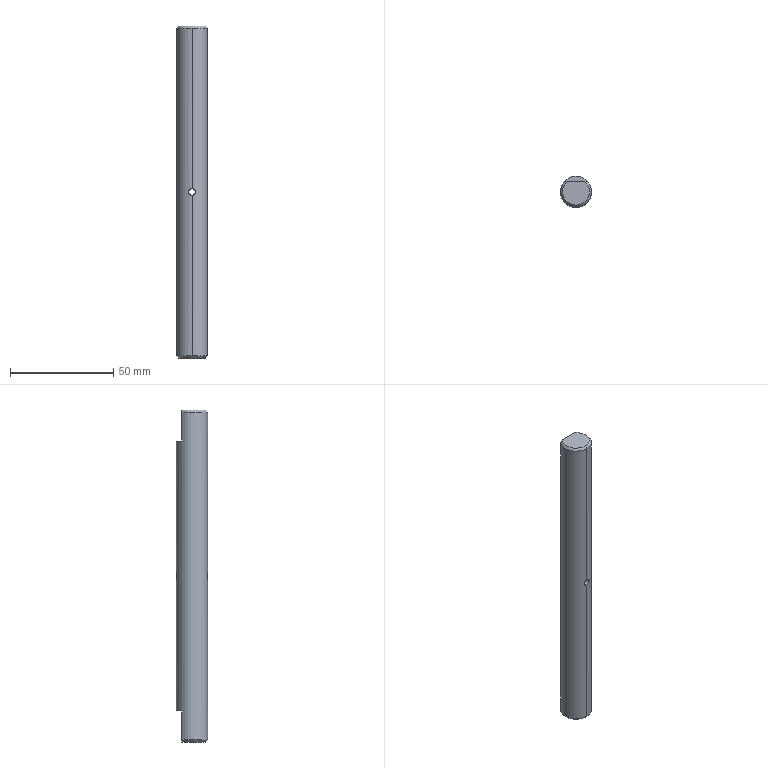Component | SolidWorks | Roller-2-1_XT-1-07-2-1 | 1 solid | 13 faces | box 15 x 15 x 160.5 mm | volume 27621 mm3 | plane 6 | cylinder 4 | cone 3 | commonest cylinder face diameters 3.3 x2 15 x2
STEP:
#1=COLOUR_RGB('',0.7922,0.8196,0.9333);
#2=FILL_AREA_STYLE_COLOUR('',#1);
#3=FILL_AREA_STYLE('',(#2));
#4=SURFACE_STYLE_FILL_AREA(#3);
#5=SURFACE_SIDE_STYLE('',(#4));
#6=SURFACE_STYLE_USAGE(.BOTH.,#5);
#7=PRESENTATION_STYLE_ASSIGNMENT((#6));
#8=CARTESIAN_POINT('',(9.421,3.972,-2.799));
#9=VERTEX_POINT('',#8);
#10=CARTESIAN_POINT('',(9.421,3.972,-2.929));
#11=VERTEX_POINT('',#10);
#12=CARTESIAN_POINT('',(9.421,3.972,-2.799));
#13=CARTESIAN_POINT('',(9.429,3.972,-2.799));
#14=CARTESIAN_POINT('',(9.438,3.972,-2.801));
#15=CARTESIAN_POINT('',(9.449,3.973,-2.806));
#16=CARTESIAN_POINT('',(9.453,3.974,-2.808));
#17=CARTESIAN_POINT('',(9.46,3.974,-2.813));
#18=CARTESIAN_POINT('',(9.464,3.975,-2.815));
#19=CARTESIAN_POINT('',(9.47,3.976,-2.821));
#20=CARTESIAN_POINT('',(9.472,3.976,-2.825));
#21=CARTESIAN_POINT('',(9.477,3.977,-2.832));
#22=CARTESIAN_POINT('',(9.479,3.978,-2.835));
#23=CARTESIAN_POINT('',(9.484,3.979,-2.847));
#24=CARTESIAN_POINT('',(9.486,3.979,-2.856));
#25=CARTESIAN_POINT('',(9.486,3.979,-2.868));
#26=CARTESIAN_POINT('',(9.485,3.979,-2.873));
#27=CARTESIAN_POINT('',(9.483,3.979,-2.881));
#28=CARTESIAN_POINT('',(9.482,3.978,-2.885));
#29=CARTESIAN_POINT('',(9.477,3.977,-2.897));
#30=CARTESIAN_POINT('',(9.473,3.976,-2.904));
#31=CARTESIAN_POINT('',(9.461,3.975,-2.916));
#32=CARTESIAN_POINT('',(9.453,3.974,-2.921));
#33=CARTESIAN_POINT('',(9.442,3.973,-2.926));
#34=CARTESIAN_POINT('',(9.438,3.972,-2.927));
#35=CARTESIAN_POINT('',(9.429,3.972,-2.929));
#36=CARTESIAN_POINT('',(9.425,3.972,-2.929));
#37=CARTESIAN_POINT('',(9.421,3.972,-2.929));
#38=B_SPLINE_CURVE_WITH_KNOTS('',3,(#12,#13,#14,#15,#16,#17,#18,#19,#20,#21,#22,#23,#24,#25,#26,#27,#28,#29,#30,#31,#32,#33,#34,#35,#36,#37),.UNSPECIFIED.,.F.,.F.,(4,2,2,2,2,2,2,2,2,2,2,2,4),(0.005175,0.005821,0.006144,0.006468,0.006791,0.007114,0.007761,0.008084,0.008408,0.009054,0.009701,0.01002,0.01035),.UNSPECIFIED.);
#39=EDGE_CURVE('',#9,#11,#38,.T.);
#40=ORIENTED_EDGE('',*,*,#39,.F.);
#41=CARTESIAN_POINT('',(9.421,4.562,-2.799));
#42=VERTEX_POINT('',#41);
#43=CARTESIAN_POINT('',(9.421,4.602,-2.799));
#44=DIRECTION('',(-0.,1.,0.));
#45=VECTOR('',#44,39.37);
#46=LINE('',#43,#45);
#47=EDGE_CURVE('',#9,#42,#46,.T.);
#48=ORIENTED_EDGE('',*,*,#47,.T.);
#49=CARTESIAN_POINT('',(9.421,4.562,-2.929));
#50=VERTEX_POINT('',#49);
#51=CARTESIAN_POINT('',(9.421,4.562,-2.929));
#52=CARTESIAN_POINT('',(9.425,4.562,-2.929));
#53=CARTESIAN_POINT('',(9.429,4.562,-2.929));
#54=CARTESIAN_POINT('',(9.437,4.562,-2.927));
#55=CARTESIAN_POINT('',(9.442,4.562,-2.926));
#56=CARTESIAN_POINT('',(9.449,4.561,-2.923));
#57=CARTESIAN_POINT('',(9.453,4.561,-2.921));
#58=CARTESIAN_POINT('',(9.46,4.56,-2.916));
#59=CARTESIAN_POINT('',(9.464,4.559,-2.913));
#60=CARTESIAN_POINT('',(9.473,4.558,-2.904));
#61=CARTESIAN_POINT('',(9.477,4.557,-2.897));
#62=CARTESIAN_POINT('',(9.484,4.556,-2.881));
#63=CARTESIAN_POINT('',(9.486,4.555,-2.873));
#64=CARTESIAN_POINT('',(9.486,4.555,-2.86));
#65=CARTESIAN_POINT('',(9.485,4.555,-2.856));
#66=CARTESIAN_POINT('',(9.483,4.556,-2.847));
#67=CARTESIAN_POINT('',(9.482,4.556,-2.843));
#68=CARTESIAN_POINT('',(9.477,4.557,-2.831));
#69=CARTESIAN_POINT('',(9.473,4.558,-2.824));
#70=CARTESIAN_POINT('',(9.464,4.559,-2.815));
#71=CARTESIAN_POINT('',(9.46,4.56,-2.813));
#72=CARTESIAN_POINT('',(9.453,4.561,-2.808));
#73=CARTESIAN_POINT('',(9.449,4.561,-2.806));
#74=CARTESIAN_POINT('',(9.442,4.562,-2.803));
#75=CARTESIAN_POINT('',(9.438,4.562,-2.801));
#76=CARTESIAN_POINT('',(9.429,4.562,-2.8));
#77=CARTESIAN_POINT('',(9.425,4.562,-2.799));
#78=CARTESIAN_POINT('',(9.421,4.562,-2.799));
#79=B_SPLINE_CURVE_WITH_KNOTS('',3,(#51,#52,#53,#54,#55,#56,#57,#58,#59,#60,#61,#62,#63,#64,#65,#66,#67,#68,#69,#70,#71,#72,#73,#74,#75,#76,#77,#78),.UNSPECIFIED.,.F.,.F.,(4,2,2,2,2,2,2,2,2,2,2,2,2,4),(0.,0.0003234,0.0006468,0.0009702,0.001294,0.00194,0.002587,0.002911,0.003234,0.003881,0.004204,0.004528,0.004851,0.005175),.UNSPECIFIED.);
#80=EDGE_CURVE('',#50,#42,#79,.T.);
#81=ORIENTED_EDGE('',*,*,#80,.F.);
#82=CARTESIAN_POINT('',(9.421,4.602,-2.929));
#83=DIRECTION('',(-0.,1.,0.));
#84=VECTOR('',#83,39.37);
#85=LINE('',#82,#84);
#86=EDGE_CURVE('',#11,#50,#85,.T.);
#87=ORIENTED_EDGE('',*,*,#86,.F.);
#88=EDGE_LOOP('',(#40,#48,#81,#87));
#89=FACE_OUTER_BOUND('',#88,.T.);
#90=CARTESIAN_POINT('',(9.421,4.602,-2.864));
#91=DIRECTION('',(-0.,1.,0.));
#92=DIRECTION('',(0.,0.,-1.));
#93=AXIS2_PLACEMENT_3D('',#90,#91,#92);
#94=CYLINDRICAL_SURFACE('',#93,0.06496);
#95=ADVANCED_FACE('',(#89),#94,.F.);
#96=CARTESIAN_POINT('',(9.421,4.011,0.2953));
#97=VERTEX_POINT('',#96);
#98=CARTESIAN_POINT('',(9.584,4.464,0.2953));
#99=VERTEX_POINT('',#98);
#100=CARTESIAN_POINT('',(9.421,4.267,0.2953));
#101=DIRECTION('',(0.,0.,1.));
#102=DIRECTION('',(0.,1.,0.));
#103=AXIS2_PLACEMENT_3D('',#100,#101,#102);
#104=CIRCLE('',#103,0.2559);
#105=EDGE_CURVE('',#97,#99,#104,.T.);
#106=ORIENTED_EDGE('',*,*,#105,.F.);
#107=CARTESIAN_POINT('',(9.421,3.972,0.2559));
#108=VERTEX_POINT('',#107);
#109=CARTESIAN_POINT('',(9.421,4.011,0.2953));
#110=DIRECTION('',(0.,-0.7071,-0.7071));
#111=VECTOR('',#110,39.37);
#112=LINE('',#109,#111);
#113=EDGE_CURVE('',#97,#108,#112,.T.);
#114=ORIENTED_EDGE('',*,*,#113,.T.);
#115=CARTESIAN_POINT('',(9.641,4.464,0.2559));
#116=VERTEX_POINT('',#115);
#117=CARTESIAN_POINT('',(9.421,4.267,0.2559));
#118=DIRECTION('',(0.,0.,-1.));
#119=DIRECTION('',(0.,1.,0.));
#120=AXIS2_PLACEMENT_3D('',#117,#118,#119);
#121=CIRCLE('',#120,0.2953);
#122=EDGE_CURVE('',#116,#108,#121,.T.);
#123=ORIENTED_EDGE('',*,*,#122,.F.);
#124=CARTESIAN_POINT('',(9.584,4.464,0.2953));
#125=CARTESIAN_POINT('',(9.603,4.464,0.2829));
#126=CARTESIAN_POINT('',(9.622,4.464,0.2696));
#127=CARTESIAN_POINT('',(9.641,4.464,0.2559));
#128=B_SPLINE_CURVE_WITH_KNOTS('',3,(#124,#125,#126,#127),.UNSPECIFIED.,.F.,.F.,(4,4),(0.,0.001751),.UNSPECIFIED.);
#129=EDGE_CURVE('',#99,#116,#128,.T.);
#130=ORIENTED_EDGE('',*,*,#129,.F.);
#131=EDGE_LOOP('',(#106,#114,#123,#130));
#132=FACE_OUTER_BOUND('',#131,.T.);
#133=CARTESIAN_POINT('',(9.421,4.267,0.2953));
#134=DIRECTION('',(0.,0.,-1.));
#135=DIRECTION('',(0.,-1.,0.));
#136=AXIS2_PLACEMENT_3D('',#133,#134,#135);
#137=CONICAL_SURFACE('',#136,0.2559,0.7854);
#138=ADVANCED_FACE('',(#132),#137,.T.);
#139=CARTESIAN_POINT('',(9.201,4.464,-0.2953));
#140=VERTEX_POINT('',#139);
#141=CARTESIAN_POINT('',(9.421,4.562,-0.2953));
#142=VERTEX_POINT('',#141);
#143=CARTESIAN_POINT('',(9.421,4.267,-0.2953));
#144=DIRECTION('',(0.,0.,-1.));
#145=DIRECTION('',(0.,-1.,0.));
#146=AXIS2_PLACEMENT_3D('',#143,#144,#145);
#147=CIRCLE('',#146,0.2953);
#148=EDGE_CURVE('',#140,#142,#147,.T.);
#149=ORIENTED_EDGE('',*,*,#148,.T.);
#150=CARTESIAN_POINT('',(9.421,4.562,0.2953));
#151=DIRECTION('',(0.,0.,-1.));
#152=VECTOR('',#151,39.37);
#153=LINE('',#150,#152);
#154=EDGE_CURVE('',#142,#42,#153,.T.);
#155=ORIENTED_EDGE('',*,*,#154,.T.);
#156=CARTESIAN_POINT('',(9.421,4.562,-2.799));
#157=CARTESIAN_POINT('',(9.412,4.562,-2.799));
#158=CARTESIAN_POINT('',(9.404,4.562,-2.801));
#159=CARTESIAN_POINT('',(9.392,4.561,-2.806));
#160=CARTESIAN_POINT('',(9.388,4.561,-2.808));
#161=CARTESIAN_POINT('',(9.381,4.56,-2.813));
#162=CARTESIAN_POINT('',(9.378,4.559,-2.815));
#163=CARTESIAN_POINT('',(9.372,4.558,-2.821));
#164=CARTESIAN_POINT('',(9.369,4.558,-2.825));
#165=CARTESIAN_POINT('',(9.364,4.557,-2.832));
#166=CARTESIAN_POINT('',(9.362,4.557,-2.835));
#167=CARTESIAN_POINT('',(9.357,4.556,-2.847));
#168=CARTESIAN_POINT('',(9.356,4.555,-2.856));
#169=CARTESIAN_POINT('',(9.356,4.555,-2.868));
#170=CARTESIAN_POINT('',(9.356,4.555,-2.873));
#171=CARTESIAN_POINT('',(9.358,4.556,-2.881));
#172=CARTESIAN_POINT('',(9.359,4.556,-2.885));
#173=CARTESIAN_POINT('',(9.364,4.557,-2.897));
#174=CARTESIAN_POINT('',(9.369,4.558,-2.904));
#175=CARTESIAN_POINT('',(9.381,4.56,-2.916));
#176=CARTESIAN_POINT('',(9.388,4.561,-2.921));
#177=CARTESIAN_POINT('',(9.4,4.562,-2.926));
#178=CARTESIAN_POINT('',(9.404,4.562,-2.927));
#179=CARTESIAN_POINT('',(9.412,4.562,-2.929));
#180=CARTESIAN_POINT('',(9.416,4.562,-2.929));
#181=CARTESIAN_POINT('',(9.421,4.562,-2.929));
#182=B_SPLINE_CURVE_WITH_KNOTS('',3,(#156,#157,#158,#159,#160,#161,#162,#163,#164,#165,#166,#167,#168,#169,#170,#171,#172,#173,#174,#175,#176,#177,#178,#179,#180,#181),.UNSPECIFIED.,.F.,.F.,(4,2,2,2,2,2,2,2,2,2,2,2,4),(0.005175,0.005821,0.006144,0.006468,0.006791,0.007114,0.007761,0.008084,0.008408,0.009054,0.009701,0.01002,0.01035),.UNSPECIFIED.);
#183=EDGE_CURVE('',#42,#50,#182,.T.);
#184=ORIENTED_EDGE('',*,*,#183,.T.);
#185=CARTESIAN_POINT('',(9.421,4.562,-5.433));
#186=VERTEX_POINT('',#185);
#187=CARTESIAN_POINT('',(9.421,4.562,0.2953));
#188=DIRECTION('',(0.,0.,-1.));
#189=VECTOR('',#188,39.37);
#190=LINE('',#187,#189);
#191=EDGE_CURVE('',#50,#186,#190,.T.);
#192=ORIENTED_EDGE('',*,*,#191,.T.);
#193=CARTESIAN_POINT('',(9.201,4.464,-5.433));
#194=VERTEX_POINT('',#193);
#195=CARTESIAN_POINT('',(9.421,4.267,-5.433));
#196=DIRECTION('',(0.,0.,1.));
#197=DIRECTION('',(0.,1.,0.));
#198=AXIS2_PLACEMENT_3D('',#195,#196,#197);
#199=CIRCLE('',#198,0.2953);
#200=EDGE_CURVE('',#186,#194,#199,.T.);
#201=ORIENTED_EDGE('',*,*,#200,.T.);
#202=CARTESIAN_POINT('',(9.201,4.464,-5.984));
#203=VERTEX_POINT('',#202);
#204=CARTESIAN_POINT('',(9.201,4.464,-5.433));
#205=DIRECTION('',(0.,0.,-1.));
#206=VECTOR('',#205,39.37);
#207=LINE('',#204,#206);
#208=EDGE_CURVE('',#194,#203,#207,.T.);
#209=ORIENTED_EDGE('',*,*,#208,.T.);
#210=CARTESIAN_POINT('',(9.421,3.972,-5.984));
#211=VERTEX_POINT('',#210);
#212=CARTESIAN_POINT('',(9.421,4.267,-5.984));
#213=DIRECTION('',(0.,0.,1.));
#214=DIRECTION('',(0.,1.,0.));
#215=AXIS2_PLACEMENT_3D('',#212,#213,#214);
#216=CIRCLE('',#215,0.2953);
#217=EDGE_CURVE('',#203,#211,#216,.T.);
#218=ORIENTED_EDGE('',*,*,#217,.T.);
#219=CARTESIAN_POINT('',(9.421,3.972,0.2953));
#220=DIRECTION('',(0.,0.,-1.));
#221=VECTOR('',#220,39.37);
#222=LINE('',#219,#221);
#223=EDGE_CURVE('',#11,#211,#222,.T.);
#224=ORIENTED_EDGE('',*,*,#223,.F.);
#225=CARTESIAN_POINT('',(9.421,3.972,-2.929));
#226=CARTESIAN_POINT('',(9.416,3.972,-2.929));
#227=CARTESIAN_POINT('',(9.412,3.972,-2.929));
#228=CARTESIAN_POINT('',(9.404,3.972,-2.927));
#229=CARTESIAN_POINT('',(9.4,3.973,-2.926));
#230=CARTESIAN_POINT('',(9.392,3.973,-2.923));
#231=CARTESIAN_POINT('',(9.388,3.974,-2.921));
#232=CARTESIAN_POINT('',(9.381,3.974,-2.916));
#233=CARTESIAN_POINT('',(9.378,3.975,-2.913));
#234=CARTESIAN_POINT('',(9.369,3.976,-2.904));
#235=CARTESIAN_POINT('',(9.364,3.977,-2.897));
#236=CARTESIAN_POINT('',(9.357,3.979,-2.881));
#237=CARTESIAN_POINT('',(9.356,3.979,-2.873));
#238=CARTESIAN_POINT('',(9.356,3.979,-2.86));
#239=CARTESIAN_POINT('',(9.356,3.979,-2.856));
#240=CARTESIAN_POINT('',(9.358,3.979,-2.847));
#241=CARTESIAN_POINT('',(9.359,3.978,-2.843));
#242=CARTESIAN_POINT('',(9.364,3.977,-2.831));
#243=CARTESIAN_POINT('',(9.369,3.976,-2.824));
#244=CARTESIAN_POINT('',(9.378,3.975,-2.815));
#245=CARTESIAN_POINT('',(9.381,3.974,-2.813));
#246=CARTESIAN_POINT('',(9.388,3.974,-2.808));
#247=CARTESIAN_POINT('',(9.392,3.973,-2.806));
#248=CARTESIAN_POINT('',(9.4,3.973,-2.803));
#249=CARTESIAN_POINT('',(9.404,3.972,-2.801));
#250=CARTESIAN_POINT('',(9.412,3.972,-2.8));
#251=CARTESIAN_POINT('',(9.416,3.972,-2.799));
#252=CARTESIAN_POINT('',(9.421,3.972,-2.799));
#253=B_SPLINE_CURVE_WITH_KNOTS('',3,(#225,#226,#227,#228,#229,#230,#231,#232,#233,#234,#235,#236,#237,#238,#239,#240,#241,#242,#243,#244,#245,#246,#247,#248,#249,#250,#251,#252),.UNSPECIFIED.,.F.,.F.,(4,2,2,2,2,2,2,2,2,2,2,2,2,4),(0.,0.0003234,0.0006468,0.0009702,0.001294,0.00194,0.002587,0.002911,0.003234,0.003881,0.004204,0.004528,0.004851,0.005175),.UNSPECIFIED.);
#254=EDGE_CURVE('',#11,#9,#253,.T.);
#255=ORIENTED_EDGE('',*,*,#254,.T.);
#256=CARTESIAN_POINT('',(9.421,3.972,0.2953));
#257=DIRECTION('',(0.,0.,-1.));
#258=VECTOR('',#257,39.37);
#259=LINE('',#256,#258);
#260=EDGE_CURVE('',#108,#9,#259,.T.);
#261=ORIENTED_EDGE('',*,*,#260,.F.);
#262=CARTESIAN_POINT('',(9.201,4.464,0.2559));
#263=VERTEX_POINT('',#262);
#264=CARTESIAN_POINT('',(9.421,4.267,0.2559));
#265=DIRECTION('',(0.,0.,-1.));
#266=DIRECTION('',(0.,1.,0.));
#267=AXIS2_PLACEMENT_3D('',#264,#265,#266);
#268=CIRCLE('',#267,0.2953);
#269=EDGE_CURVE('',#108,#263,#268,.T.);
#270=ORIENTED_EDGE('',*,*,#269,.T.);
#271=CARTESIAN_POINT('',(9.201,4.464,-0.2953));
#272=DIRECTION('',(0.,0.,1.));
#273=VECTOR('',#272,39.37);
#274=LINE('',#271,#273);
#275=EDGE_CURVE('',#140,#263,#274,.T.);
#276=ORIENTED_EDGE('',*,*,#275,.F.);
#277=EDGE_LOOP('',(#149,#155,#184,#192,#201,#209,#218,#224,#255,#261,#270,#276));
#278=FACE_OUTER_BOUND('',#277,.T.);
#279=CARTESIAN_POINT('',(9.421,4.267,0.2953));
#280=DIRECTION('',(0.,0.,-1.));
#281=DIRECTION('',(0.,-1.,0.));
#282=AXIS2_PLACEMENT_3D('',#279,#280,#281);
#283=CYLINDRICAL_SURFACE('',#282,0.2953);
#284=ADVANCED_FACE('',(#278),#283,.T.);
#285=ORIENTED_EDGE('',*,*,#154,.F.);
#286=CARTESIAN_POINT('',(9.641,4.464,-0.2953));
#287=VERTEX_POINT('',#286);
#288=CARTESIAN_POINT('',(9.421,4.267,-0.2953));
#289=DIRECTION('',(0.,0.,-1.));
#290=DIRECTION('',(0.,-1.,0.));
#291=AXIS2_PLACEMENT_3D('',#288,#289,#290);
#292=CIRCLE('',#291,0.2953);
#293=EDGE_CURVE('',#142,#287,#292,.T.);
#294=ORIENTED_EDGE('',*,*,#293,.T.);
#295=CARTESIAN_POINT('',(9.641,4.464,-0.2953));
#296=DIRECTION('',(0.,0.,1.));
#297=VECTOR('',#296,39.37);
#298=LINE('',#295,#297);
#299=EDGE_CURVE('',#287,#116,#298,.T.);
#300=ORIENTED_EDGE('',*,*,#299,.T.);
#301=ORIENTED_EDGE('',*,*,#122,.T.);
#302=ORIENTED_EDGE('',*,*,#260,.T.);
#303=ORIENTED_EDGE('',*,*,#39,.T.);
#304=ORIENTED_EDGE('',*,*,#223,.T.);
#305=CARTESIAN_POINT('',(9.641,4.464,-5.984));
#306=VERTEX_POINT('',#305);
#307=CARTESIAN_POINT('',(9.421,4.267,-5.984));
#308=DIRECTION('',(0.,0.,1.));
#309=DIRECTION('',(0.,1.,0.));
#310=AXIS2_PLACEMENT_3D('',#307,#308,#309);
#311=CIRCLE('',#310,0.2953);
#312=EDGE_CURVE('',#211,#306,#311,.T.);
#313=ORIENTED_EDGE('',*,*,#312,.T.);
#314=CARTESIAN_POINT('',(9.641,4.464,-5.433));
#315=VERTEX_POINT('',#314);
#316=CARTESIAN_POINT('',(9.641,4.464,-5.433));
#317=DIRECTION('',(0.,0.,-1.));
#318=VECTOR('',#317,39.37);
#319=LINE('',#316,#318);
#320=EDGE_CURVE('',#315,#306,#319,.T.);
#321=ORIENTED_EDGE('',*,*,#320,.F.);
#322=CARTESIAN_POINT('',(9.421,4.267,-5.433));
#323=DIRECTION('',(0.,0.,1.));
#324=DIRECTION('',(0.,1.,0.));
#325=AXIS2_PLACEMENT_3D('',#322,#323,#324);
#326=CIRCLE('',#325,0.2953);
#327=EDGE_CURVE('',#315,#186,#326,.T.);
#328=ORIENTED_EDGE('',*,*,#327,.T.);
#329=ORIENTED_EDGE('',*,*,#191,.F.);
#330=ORIENTED_EDGE('',*,*,#80,.T.);
#331=EDGE_LOOP('',(#285,#294,#300,#301,#302,#303,#304,#313,#321,#328,#329,#330));
#332=FACE_OUTER_BOUND('',#331,.T.);
#333=CARTESIAN_POINT('',(9.421,4.267,0.2953));
#334=DIRECTION('',(0.,0.,-1.));
#335=DIRECTION('',(0.,-1.,0.));
#336=AXIS2_PLACEMENT_3D('',#333,#334,#335);
#337=CYLINDRICAL_SURFACE('',#336,0.2953);
#338=ADVANCED_FACE('',(#332),#337,.T.);
#339=CARTESIAN_POINT('',(9.257,4.464,0.2953));
#340=VERTEX_POINT('',#339);
#341=CARTESIAN_POINT('',(9.201,4.464,0.2953));
#342=DIRECTION('',(1.,0.,0.));
#343=VECTOR('',#342,39.37);
#344=LINE('',#341,#343);
#345=EDGE_CURVE('',#340,#99,#344,.T.);
#346=ORIENTED_EDGE('',*,*,#345,.F.);
#347=CARTESIAN_POINT('',(9.421,4.267,0.2953));
#348=DIRECTION('',(0.,0.,1.));
#349=DIRECTION('',(0.,1.,0.));
#350=AXIS2_PLACEMENT_3D('',#347,#348,#349);
#351=CIRCLE('',#350,0.2559);
#352=EDGE_CURVE('',#340,#97,#351,.T.);
#353=ORIENTED_EDGE('',*,*,#352,.T.);
#354=ORIENTED_EDGE('',*,*,#105,.T.);
#355=EDGE_LOOP('',(#346,#353,#354));
#356=FACE_OUTER_BOUND('',#355,.T.);
#357=CARTESIAN_POINT('',(9.421,4.267,0.2953));
#358=DIRECTION('',(0.,0.,1.));
#359=DIRECTION('',(-0.,1.,0.));
#360=AXIS2_PLACEMENT_3D('',#357,#358,#359);
#361=PLANE('',#360);
#362=ADVANCED_FACE('',(#356),#361,.T.);
#363=CARTESIAN_POINT('',(9.584,4.464,-6.024));
#364=VERTEX_POINT('',#363);
#365=CARTESIAN_POINT('',(9.257,4.464,-6.024));
#366=VERTEX_POINT('',#365);
#367=CARTESIAN_POINT('',(9.201,4.464,-6.024));
#368=DIRECTION('',(-1.,-0.,0.));
#369=VECTOR('',#368,39.37);
#370=LINE('',#367,#369);
#371=EDGE_CURVE('',#364,#366,#370,.T.);
#372=ORIENTED_EDGE('',*,*,#371,.F.);
#373=CARTESIAN_POINT('',(9.421,4.267,-6.024));
#374=DIRECTION('',(0.,0.,-1.));
#375=DIRECTION('',(0.,1.,0.));
#376=AXIS2_PLACEMENT_3D('',#373,#374,#375);
#377=CIRCLE('',#376,0.2559);
#378=EDGE_CURVE('',#364,#366,#377,.T.);
#379=ORIENTED_EDGE('',*,*,#378,.T.);
#380=EDGE_LOOP('',(#372,#379));
#381=FACE_OUTER_BOUND('',#380,.T.);
#382=CARTESIAN_POINT('',(9.421,4.267,-6.024));
#383=DIRECTION('',(0.,0.,1.));
#384=DIRECTION('',(-0.,1.,0.));
#385=AXIS2_PLACEMENT_3D('',#382,#383,#384);
#386=PLANE('',#385);
#387=ADVANCED_FACE('',(#381),#386,.F.);
#388=CARTESIAN_POINT('',(9.201,4.464,-0.2953));
#389=DIRECTION('',(1.,0.,0.));
#390=VECTOR('',#389,39.37);
#391=LINE('',#388,#390);
#392=EDGE_CURVE('',#140,#287,#391,.T.);
#393=ORIENTED_EDGE('',*,*,#392,.T.);
#394=ORIENTED_EDGE('',*,*,#293,.F.);
#395=ORIENTED_EDGE('',*,*,#148,.F.);
#396=EDGE_LOOP('',(#393,#394,#395));
#397=FACE_OUTER_BOUND('',#396,.T.);
#398=CARTESIAN_POINT('',(9.201,4.728,-0.2953));
#399=DIRECTION('',(0.,0.,-1.));
#400=DIRECTION('',(0.,-1.,0.));
#401=AXIS2_PLACEMENT_3D('',#398,#399,#400);
#402=PLANE('',#401);
#403=ADVANCED_FACE('',(#397),#402,.F.);
#404=ORIENTED_EDGE('',*,*,#345,.T.);
#405=ORIENTED_EDGE('',*,*,#129,.T.);
#406=ORIENTED_EDGE('',*,*,#299,.F.);
#407=ORIENTED_EDGE('',*,*,#392,.F.);
#408=ORIENTED_EDGE('',*,*,#275,.T.);
#409=CARTESIAN_POINT('',(9.201,4.464,0.2559));
#410=CARTESIAN_POINT('',(9.219,4.464,0.2696));
#411=CARTESIAN_POINT('',(9.238,4.464,0.2829));
#412=CARTESIAN_POINT('',(9.257,4.464,0.2953));
#413=B_SPLINE_CURVE_WITH_KNOTS('',3,(#409,#410,#411,#412),.UNSPECIFIED.,.F.,.F.,(4,4),(0.,0.001751),.UNSPECIFIED.);
#414=EDGE_CURVE('',#263,#340,#413,.T.);
#415=ORIENTED_EDGE('',*,*,#414,.T.);
#416=EDGE_LOOP('',(#404,#405,#406,#407,#408,#415));
#417=FACE_OUTER_BOUND('',#416,.T.);
#418=CARTESIAN_POINT('',(9.201,4.464,-0.2953));
#419=DIRECTION('',(0.,-1.,0.));
#420=DIRECTION('',(0.,0.,1.));
#421=AXIS2_PLACEMENT_3D('',#418,#419,#420);
#422=PLANE('',#421);
#423=ADVANCED_FACE('',(#417),#422,.F.);
#424=CARTESIAN_POINT('',(9.201,4.464,-5.433));
#425=DIRECTION('',(-1.,-0.,0.));
#426=VECTOR('',#425,39.37);
#427=LINE('',#424,#426);
#428=EDGE_CURVE('',#315,#194,#427,.T.);
#429=ORIENTED_EDGE('',*,*,#428,.T.);
#430=ORIENTED_EDGE('',*,*,#200,.F.);
#431=ORIENTED_EDGE('',*,*,#327,.F.);
#432=EDGE_LOOP('',(#429,#430,#431));
#433=FACE_OUTER_BOUND('',#432,.T.);
#434=CARTESIAN_POINT('',(9.201,4.464,-5.433));
#435=DIRECTION('',(0.,0.,1.));
#436=DIRECTION('',(-0.,1.,0.));
#437=AXIS2_PLACEMENT_3D('',#434,#435,#436);
#438=PLANE('',#437);
#439=ADVANCED_FACE('',(#433),#438,.F.);
#440=ORIENTED_EDGE('',*,*,#320,.T.);
#441=CARTESIAN_POINT('',(9.641,4.464,-5.984));
#442=CARTESIAN_POINT('',(9.622,4.464,-5.998));
#443=CARTESIAN_POINT('',(9.603,4.464,-6.011));
#444=CARTESIAN_POINT('',(9.584,4.464,-6.024));
#445=B_SPLINE_CURVE_WITH_KNOTS('',3,(#441,#442,#443,#444),.UNSPECIFIED.,.F.,.F.,(4,4),(0.,0.001751),.UNSPECIFIED.);
#446=EDGE_CURVE('',#306,#364,#445,.T.);
#447=ORIENTED_EDGE('',*,*,#446,.T.);
#448=ORIENTED_EDGE('',*,*,#371,.T.);
#449=CARTESIAN_POINT('',(9.257,4.464,-6.024));
#450=CARTESIAN_POINT('',(9.238,4.464,-6.011));
#451=CARTESIAN_POINT('',(9.219,4.464,-5.998));
#452=CARTESIAN_POINT('',(9.201,4.464,-5.984));
#453=B_SPLINE_CURVE_WITH_KNOTS('',3,(#449,#450,#451,#452),.UNSPECIFIED.,.F.,.F.,(4,4),(0.,0.001751),.UNSPECIFIED.);
#454=EDGE_CURVE('',#366,#203,#453,.T.);
#455=ORIENTED_EDGE('',*,*,#454,.T.);
#456=ORIENTED_EDGE('',*,*,#208,.F.);
#457=ORIENTED_EDGE('',*,*,#428,.F.);
#458=EDGE_LOOP('',(#440,#447,#448,#455,#456,#457));
#459=FACE_OUTER_BOUND('',#458,.T.);
#460=CARTESIAN_POINT('',(9.201,4.464,-5.433));
#461=DIRECTION('',(0.,-1.,0.));
#462=DIRECTION('',(0.,0.,1.));
#463=AXIS2_PLACEMENT_3D('',#460,#461,#462);
#464=PLANE('',#463);
#465=ADVANCED_FACE('',(#459),#464,.F.);
#466=ORIENTED_EDGE('',*,*,#454,.F.);
#467=ORIENTED_EDGE('',*,*,#378,.F.);
#468=ORIENTED_EDGE('',*,*,#446,.F.);
#469=ORIENTED_EDGE('',*,*,#312,.F.);
#470=ORIENTED_EDGE('',*,*,#217,.F.);
#471=EDGE_LOOP('',(#466,#467,#468,#469,#470));
#472=FACE_OUTER_BOUND('',#471,.T.);
#473=CARTESIAN_POINT('',(9.421,4.267,-5.984));
#474=DIRECTION('',(0.,0.,1.));
#475=DIRECTION('',(0.,1.,0.));
#476=AXIS2_PLACEMENT_3D('',#473,#474,#475);
#477=CONICAL_SURFACE('',#476,0.2953,0.7854);
#478=ADVANCED_FACE('',(#472),#477,.T.);
#479=ORIENTED_EDGE('',*,*,#113,.F.);
#480=ORIENTED_EDGE('',*,*,#352,.F.);
#481=ORIENTED_EDGE('',*,*,#414,.F.);
#482=ORIENTED_EDGE('',*,*,#269,.F.);
#483=EDGE_LOOP('',(#479,#480,#481,#482));
#484=FACE_OUTER_BOUND('',#483,.T.);
#485=CARTESIAN_POINT('',(9.421,4.267,0.2953));
#486=DIRECTION('',(0.,0.,-1.));
#487=DIRECTION('',(0.,-1.,0.));
#488=AXIS2_PLACEMENT_3D('',#485,#486,#487);
#489=CONICAL_SURFACE('',#488,0.2559,0.7854);
#490=ADVANCED_FACE('',(#484),#489,.T.);
#491=ORIENTED_EDGE('',*,*,#47,.F.);
#492=ORIENTED_EDGE('',*,*,#254,.F.);
#493=ORIENTED_EDGE('',*,*,#86,.T.);
#494=ORIENTED_EDGE('',*,*,#183,.F.);
#495=EDGE_LOOP('',(#491,#492,#493,#494));
#496=FACE_OUTER_BOUND('',#495,.T.);
#497=CARTESIAN_POINT('',(9.421,4.602,-2.864));
#498=DIRECTION('',(-0.,1.,0.));
#499=DIRECTION('',(0.,0.,-1.));
#500=AXIS2_PLACEMENT_3D('',#497,#498,#499);
#501=CYLINDRICAL_SURFACE('',#500,0.06496);
#502=ADVANCED_FACE('',(#496),#501,.F.);
#503=CLOSED_SHELL('',(#95,#138,#284,#338,#362,#387,#403,#423,#439,#465,#478,#490,#502));
#504=MANIFOLD_SOLID_BREP('',#503);
#505=STYLED_ITEM('',(#7),#504);
#506=(LENGTH_UNIT()NAMED_UNIT(*)SI_UNIT($,.METRE.));
#507=LENGTH_MEASURE_WITH_UNIT(LENGTH_MEASURE(0.0254),#506);
#508=DIMENSIONAL_EXPONENTS(1.,0.,0.,0.,0.,0.,0.);
#509=(CONVERSION_BASED_UNIT('',#507)LENGTH_UNIT()NAMED_UNIT(#508));
#510=UNCERTAINTY_MEASURE_WITH_UNIT(LENGTH_MEASURE(0.00001),#509,'','');
#511=(NAMED_UNIT(*)PLANE_ANGLE_UNIT()SI_UNIT($,.RADIAN.));
#512=(NAMED_UNIT(*)SI_UNIT($,.STERADIAN.)SOLID_ANGLE_UNIT());
#513=(GEOMETRIC_REPRESENTATION_CONTEXT(3)GLOBAL_UNCERTAINTY_ASSIGNED_CONTEXT((#510))GLOBAL_UNIT_ASSIGNED_CONTEXT((#509,#511,#512))REPRESENTATION_CONTEXT('',''));
#514=MECHANICAL_DESIGN_GEOMETRIC_PRESENTATION_REPRESENTATION('',(#505),#513);
#515=CARTESIAN_POINT('',(0.,0.,0.));
#516=DIRECTION('',(0.,0.,1.));
#517=DIRECTION('',(1.,0.,0.));
#518=AXIS2_PLACEMENT_3D('',#515,#516,#517);
#519=(LENGTH_UNIT()NAMED_UNIT(*)SI_UNIT($,.METRE.));
#520=LENGTH_MEASURE_WITH_UNIT(LENGTH_MEASURE(0.0254),#519);
#521=DIMENSIONAL_EXPONENTS(1.,0.,0.,0.,0.,0.,0.);
#522=(CONVERSION_BASED_UNIT('',#520)LENGTH_UNIT()NAMED_UNIT(#521));
#523=UNCERTAINTY_MEASURE_WITH_UNIT(LENGTH_MEASURE(0.00001),#522,'','');
#524=(NAMED_UNIT(*)PLANE_ANGLE_UNIT()SI_UNIT($,.RADIAN.));
#525=(NAMED_UNIT(*)SI_UNIT($,.STERADIAN.)SOLID_ANGLE_UNIT());
#526=(GEOMETRIC_REPRESENTATION_CONTEXT(3)GLOBAL_UNCERTAINTY_ASSIGNED_CONTEXT((#523))GLOBAL_UNIT_ASSIGNED_CONTEXT((#522,#524,#525))REPRESENTATION_CONTEXT('',''));
#527=ADVANCED_BREP_SHAPE_REPRESENTATION('',(#504,#518),#526);
#528=PRESENTATION_LAYER_ASSIGNMENT('','',(#505));